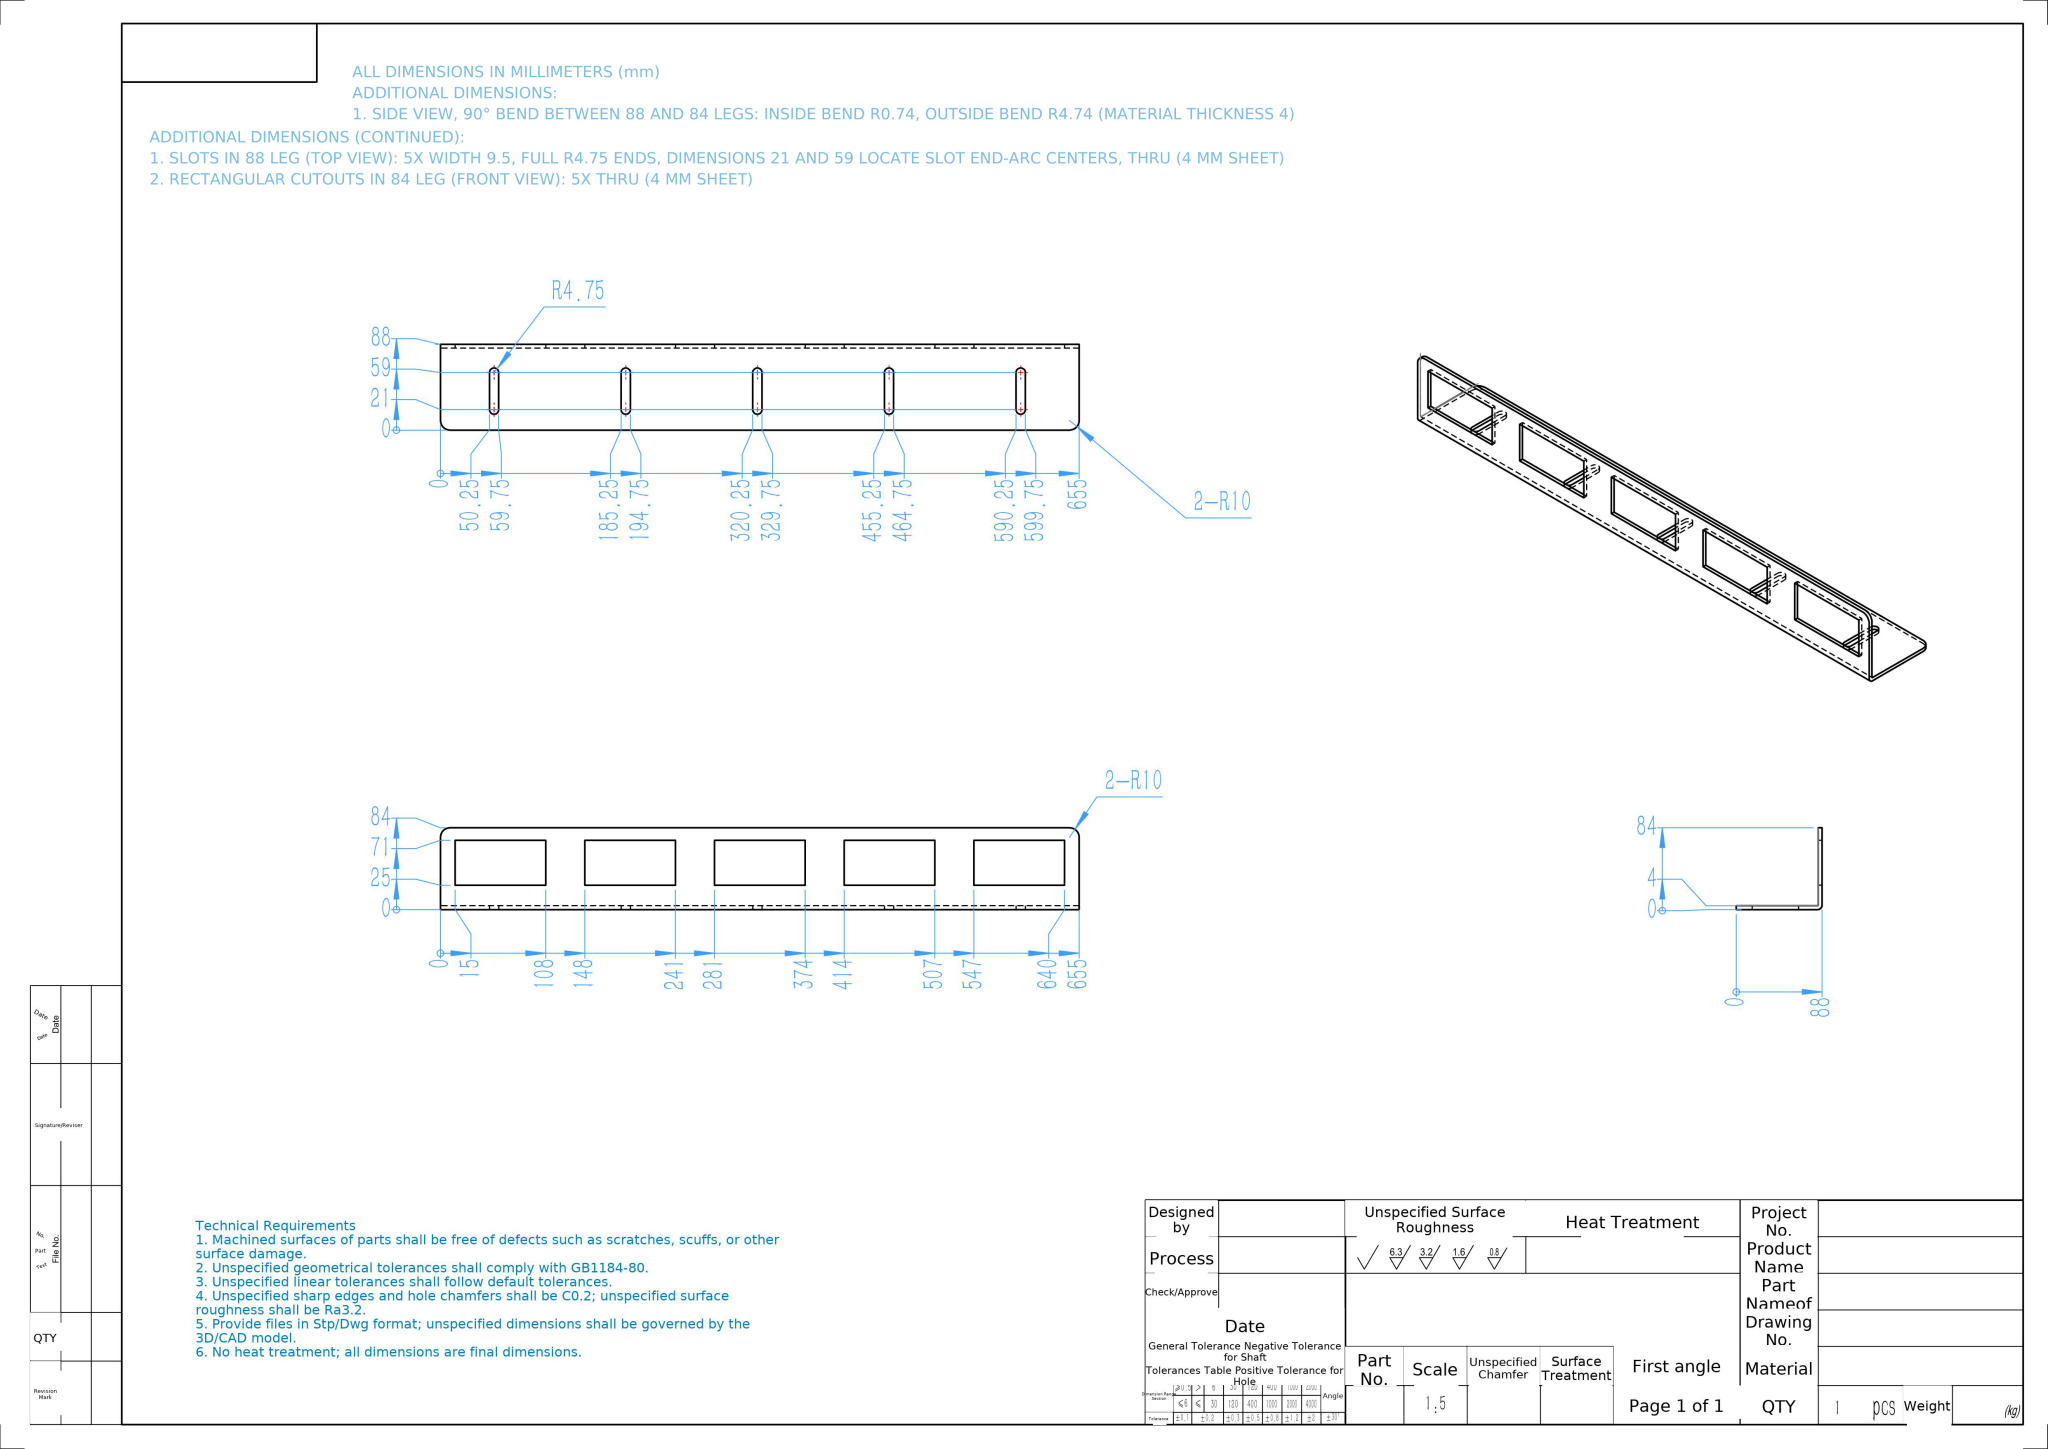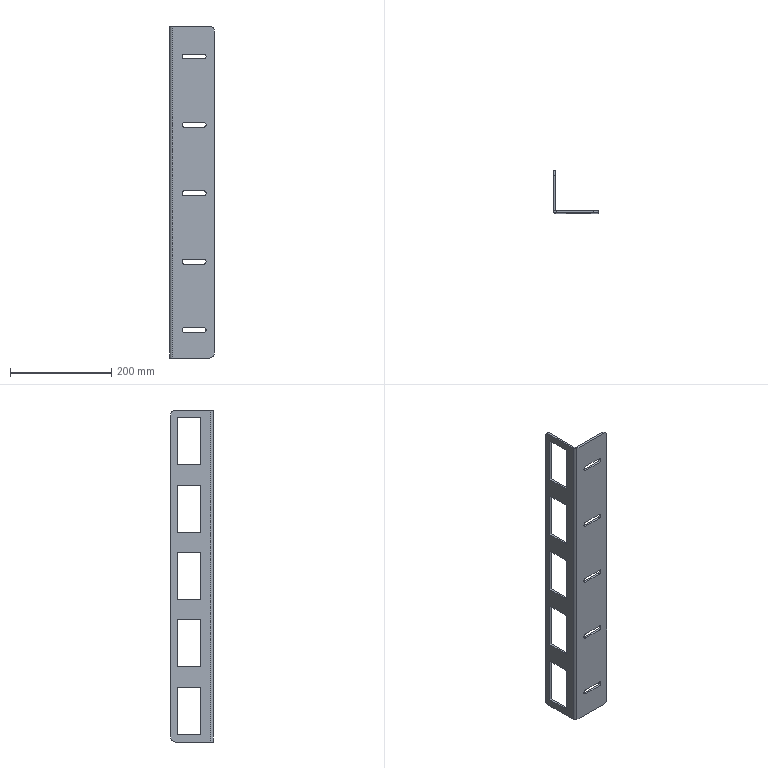Part | NX | mm | 1 solid | 58 faces | box 88 x 84 x 655 mm | volume 342542 mm3 | plane 42 | cylinder 16 | commonest cylinder face diameters 9.5 x10 20 x4 1.473 x1 9.473 x1